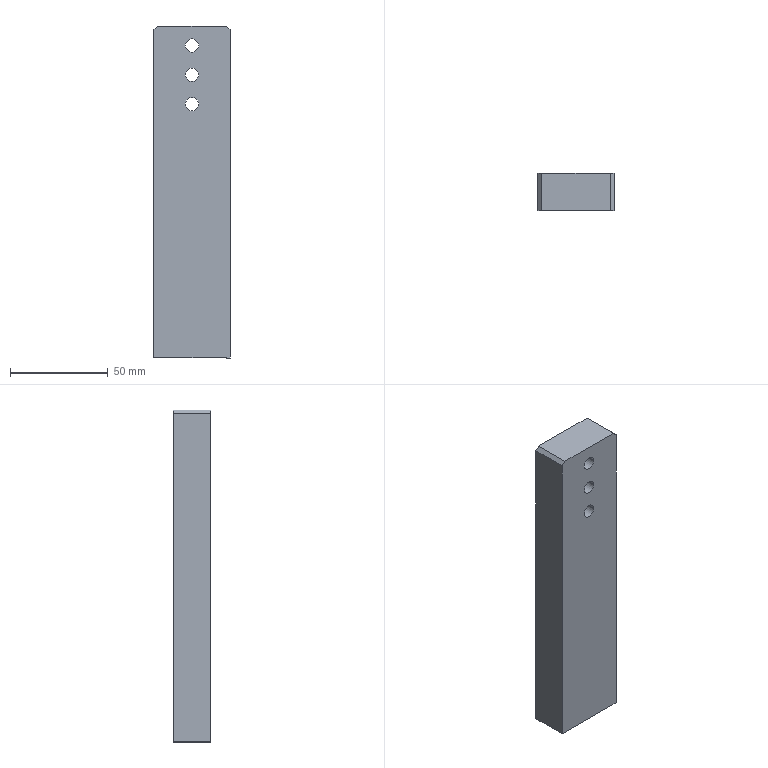Component | SolidWorks | FixedBlock-1 | 1 solid | 22 faces | box 39 x 19 x 170 mm | volume 123215 mm3 | cylinder 10 | plane 8 | cone 4 | commonest cylinder face diameters 6.8 x6 5 x4
build123d program:
from build123d import *

# Parameters (mm, degrees)
SKETCH2_W             = 39
SKETCH2_H             = 170
BOSS_EXTRUDE1_DEPTH   = 19
M6_TAPPED_HOLE1_D     = 5
M6_TAPPED_HOLE1_DEPTH = 15
M6_TAPPED_HOLE1_TIP   = 1.502
M8_TAPPED_HOLE1_D     = 6.8
M8_TAPPED_HOLE1_DEPTH = 19.75
M8_TAPPED_HOLE1_TIP   = 2.043
CHAMFER1_SIZE         = 2


with BuildPart() as part:
    # Sketch2 → Boss-Extrude1 (new body)
    with BuildSketch(Plane.XY):
        Rectangle(SKETCH2_W, SKETCH2_H)
    extrude(amount=BOSS_EXTRUDE1_DEPTH)

    # M6 Tapped Hole1
    with Locations(Plane(origin=(10, -85, 9.5), x_dir=(0, 0, -1), z_dir=(0, -1, 0))):
        with Locations((0, 0), (0, -20)):
            Hole(M6_TAPPED_HOLE1_D / 2, depth=M6_TAPPED_HOLE1_DEPTH)
            with Locations((0, 0, -(M6_TAPPED_HOLE1_DEPTH + M6_TAPPED_HOLE1_TIP / 2))):  # 118° drill point
                Cone(0, M6_TAPPED_HOLE1_D / 2, M6_TAPPED_HOLE1_TIP, mode=Mode.SUBTRACT)

    # M8 Tapped Hole1
    with Locations(Plane(origin=(0, 45, 19), x_dir=(1, 0, 0), z_dir=(0, 0, 1))):
        with Locations((0, 0), (0, 15), (0, 30)):
            Hole(M8_TAPPED_HOLE1_D / 2, depth=M8_TAPPED_HOLE1_DEPTH)
            with Locations((0, 0, -(M8_TAPPED_HOLE1_DEPTH + M8_TAPPED_HOLE1_TIP / 2))):  # 118° drill point
                Cone(0, M8_TAPPED_HOLE1_D / 2, M8_TAPPED_HOLE1_TIP, mode=Mode.SUBTRACT)

    # Chamfer1
    chamfer1_edges = [part.edges().sort_by_distance(p)[0] for p in [
        (-19.5, 85, 9.5),
        (19.5, 85, 9.5),
    ]]
    chamfer(chamfer1_edges, length=CHAMFER1_SIZE)


solid = part.part

# Placed as in the assembly
solid = solid.moved(Location((-48.047, 15.46, 106), (90, 0, 0)))
STEP:
#1=COLOUR_RGB('',0.7922,0.8196,0.9333);
#2=FILL_AREA_STYLE_COLOUR('',#1);
#3=FILL_AREA_STYLE('',(#2));
#4=SURFACE_STYLE_FILL_AREA(#3);
#5=SURFACE_SIDE_STYLE('',(#4));
#6=SURFACE_STYLE_USAGE(.BOTH.,#5);
#7=PRESENTATION_STYLE_ASSIGNMENT((#6));
#8=CARTESIAN_POINT('',(-1.758,0.6087,5.945));
#9=VERTEX_POINT('',#8);
#10=CARTESIAN_POINT('',(-2.025,0.6087,5.945));
#11=VERTEX_POINT('',#10);
#12=CARTESIAN_POINT('',(-1.892,0.6087,5.945));
#13=DIRECTION('',(-0.,1.,0.));
#14=DIRECTION('',(-1.,-0.,0.));
#15=AXIS2_PLACEMENT_3D('',#12,#13,#14);
#16=CIRCLE('',#15,0.1339);
#17=EDGE_CURVE('',#9,#11,#16,.T.);
#18=ORIENTED_EDGE('',*,*,#17,.T.);
#19=CARTESIAN_POINT('',(-2.025,-0.1394,5.945));
#20=VERTEX_POINT('',#19);
#21=CARTESIAN_POINT('',(-2.025,-0.1394,5.945));
#22=DIRECTION('',(0.,-1.,-0.));
#23=VECTOR('',#22,39.37);
#24=LINE('',#21,#23);
#25=EDGE_CURVE('',#11,#20,#24,.T.);
#26=ORIENTED_EDGE('',*,*,#25,.T.);
#27=CARTESIAN_POINT('',(-1.758,-0.1394,5.945));
#28=VERTEX_POINT('',#27);
#29=CARTESIAN_POINT('',(-1.892,-0.1394,5.945));
#30=DIRECTION('',(0.,-1.,-0.));
#31=DIRECTION('',(1.,0.,-0.));
#32=AXIS2_PLACEMENT_3D('',#29,#30,#31);
#33=CIRCLE('',#32,0.1339);
#34=EDGE_CURVE('',#20,#28,#33,.T.);
#35=ORIENTED_EDGE('',*,*,#34,.T.);
#36=CARTESIAN_POINT('',(-1.758,-0.1394,5.945));
#37=DIRECTION('',(0.,-1.,-0.));
#38=VECTOR('',#37,39.37);
#39=LINE('',#36,#38);
#40=EDGE_CURVE('',#9,#28,#39,.T.);
#41=ORIENTED_EDGE('',*,*,#40,.F.);
#42=EDGE_LOOP('',(#18,#26,#35,#41));
#43=FACE_OUTER_BOUND('',#42,.T.);
#44=CARTESIAN_POINT('',(-1.892,-0.1394,5.945));
#45=DIRECTION('',(0.,-1.,-0.));
#46=DIRECTION('',(1.,0.,-0.));
#47=AXIS2_PLACEMENT_3D('',#44,#45,#46);
#48=CYLINDRICAL_SURFACE('',#47,0.1339);
#49=ADVANCED_FACE('',(#43),#48,.F.);
#50=CARTESIAN_POINT('',(-1.758,0.6087,6.535));
#51=VERTEX_POINT('',#50);
#52=CARTESIAN_POINT('',(-2.025,0.6087,6.535));
#53=VERTEX_POINT('',#52);
#54=CARTESIAN_POINT('',(-1.892,0.6087,6.535));
#55=DIRECTION('',(-0.,1.,0.));
#56=DIRECTION('',(-1.,-0.,0.));
#57=AXIS2_PLACEMENT_3D('',#54,#55,#56);
#58=CIRCLE('',#57,0.1339);
#59=EDGE_CURVE('',#51,#53,#58,.T.);
#60=ORIENTED_EDGE('',*,*,#59,.T.);
#61=CARTESIAN_POINT('',(-2.025,-0.1394,6.535));
#62=VERTEX_POINT('',#61);
#63=CARTESIAN_POINT('',(-2.025,-0.1394,6.535));
#64=DIRECTION('',(0.,-1.,-0.));
#65=VECTOR('',#64,39.37);
#66=LINE('',#63,#65);
#67=EDGE_CURVE('',#53,#62,#66,.T.);
#68=ORIENTED_EDGE('',*,*,#67,.T.);
#69=CARTESIAN_POINT('',(-1.758,-0.1394,6.535));
#70=VERTEX_POINT('',#69);
#71=CARTESIAN_POINT('',(-1.892,-0.1394,6.535));
#72=DIRECTION('',(0.,-1.,-0.));
#73=DIRECTION('',(1.,0.,-0.));
#74=AXIS2_PLACEMENT_3D('',#71,#72,#73);
#75=CIRCLE('',#74,0.1339);
#76=EDGE_CURVE('',#62,#70,#75,.T.);
#77=ORIENTED_EDGE('',*,*,#76,.T.);
#78=CARTESIAN_POINT('',(-1.758,-0.1394,6.535));
#79=DIRECTION('',(0.,-1.,-0.));
#80=VECTOR('',#79,39.37);
#81=LINE('',#78,#80);
#82=EDGE_CURVE('',#51,#70,#81,.T.);
#83=ORIENTED_EDGE('',*,*,#82,.F.);
#84=EDGE_LOOP('',(#60,#68,#77,#83));
#85=FACE_OUTER_BOUND('',#84,.T.);
#86=CARTESIAN_POINT('',(-1.892,-0.1394,6.535));
#87=DIRECTION('',(0.,-1.,-0.));
#88=DIRECTION('',(1.,0.,-0.));
#89=AXIS2_PLACEMENT_3D('',#86,#87,#88);
#90=CYLINDRICAL_SURFACE('',#89,0.1339);
#91=ADVANCED_FACE('',(#85),#90,.F.);
#92=CARTESIAN_POINT('',(-1.758,0.6087,7.126));
#93=VERTEX_POINT('',#92);
#94=CARTESIAN_POINT('',(-2.025,0.6087,7.126));
#95=VERTEX_POINT('',#94);
#96=CARTESIAN_POINT('',(-1.892,0.6087,7.126));
#97=DIRECTION('',(-0.,1.,0.));
#98=DIRECTION('',(-1.,-0.,0.));
#99=AXIS2_PLACEMENT_3D('',#96,#97,#98);
#100=CIRCLE('',#99,0.1339);
#101=EDGE_CURVE('',#93,#95,#100,.T.);
#102=ORIENTED_EDGE('',*,*,#101,.T.);
#103=CARTESIAN_POINT('',(-2.025,-0.1394,7.126));
#104=VERTEX_POINT('',#103);
#105=CARTESIAN_POINT('',(-2.025,-0.1394,7.126));
#106=DIRECTION('',(0.,-1.,-0.));
#107=VECTOR('',#106,39.37);
#108=LINE('',#105,#107);
#109=EDGE_CURVE('',#95,#104,#108,.T.);
#110=ORIENTED_EDGE('',*,*,#109,.T.);
#111=CARTESIAN_POINT('',(-1.758,-0.1394,7.126));
#112=VERTEX_POINT('',#111);
#113=CARTESIAN_POINT('',(-1.892,-0.1394,7.126));
#114=DIRECTION('',(0.,-1.,-0.));
#115=DIRECTION('',(1.,0.,-0.));
#116=AXIS2_PLACEMENT_3D('',#113,#114,#115);
#117=CIRCLE('',#116,0.1339);
#118=EDGE_CURVE('',#104,#112,#117,.T.);
#119=ORIENTED_EDGE('',*,*,#118,.T.);
#120=CARTESIAN_POINT('',(-1.758,-0.1394,7.126));
#121=DIRECTION('',(0.,-1.,-0.));
#122=VECTOR('',#121,39.37);
#123=LINE('',#120,#122);
#124=EDGE_CURVE('',#93,#112,#123,.T.);
#125=ORIENTED_EDGE('',*,*,#124,.F.);
#126=EDGE_LOOP('',(#102,#110,#119,#125));
#127=FACE_OUTER_BOUND('',#126,.T.);
#128=CARTESIAN_POINT('',(-1.892,-0.1394,7.126));
#129=DIRECTION('',(0.,-1.,-0.));
#130=DIRECTION('',(1.,0.,-0.));
#131=AXIS2_PLACEMENT_3D('',#128,#129,#130);
#132=CYLINDRICAL_SURFACE('',#131,0.1339);
#133=ADVANCED_FACE('',(#127),#132,.F.);
#134=CARTESIAN_POINT('',(-1.498,0.1362,1.417));
#135=VERTEX_POINT('',#134);
#136=CARTESIAN_POINT('',(-1.498,0.3331,1.417));
#137=VERTEX_POINT('',#136);
#138=CARTESIAN_POINT('',(-1.498,0.2347,1.417));
#139=DIRECTION('',(-0.,0.,-1.));
#140=DIRECTION('',(0.,1.,0.));
#141=AXIS2_PLACEMENT_3D('',#138,#139,#140);
#142=CIRCLE('',#141,0.09843);
#143=EDGE_CURVE('',#135,#137,#142,.T.);
#144=ORIENTED_EDGE('',*,*,#143,.F.);
#145=CARTESIAN_POINT('',(-1.498,0.1362,0.8268));
#146=VERTEX_POINT('',#145);
#147=CARTESIAN_POINT('',(-1.498,0.1362,0.8268));
#148=DIRECTION('',(-0.,0.,-1.));
#149=VECTOR('',#148,39.37);
#150=LINE('',#147,#149);
#151=EDGE_CURVE('',#135,#146,#150,.T.);
#152=ORIENTED_EDGE('',*,*,#151,.T.);
#153=CARTESIAN_POINT('',(-1.498,0.3331,0.8268));
#154=VERTEX_POINT('',#153);
#155=CARTESIAN_POINT('',(-1.498,0.2347,0.8268));
#156=DIRECTION('',(-0.,0.,-1.));
#157=DIRECTION('',(0.,1.,0.));
#158=AXIS2_PLACEMENT_3D('',#155,#156,#157);
#159=CIRCLE('',#158,0.09843);
#160=EDGE_CURVE('',#146,#154,#159,.T.);
#161=ORIENTED_EDGE('',*,*,#160,.T.);
#162=CARTESIAN_POINT('',(-1.498,0.3331,0.8268));
#163=DIRECTION('',(-0.,0.,-1.));
#164=VECTOR('',#163,39.37);
#165=LINE('',#162,#164);
#166=EDGE_CURVE('',#137,#154,#165,.T.);
#167=ORIENTED_EDGE('',*,*,#166,.F.);
#168=EDGE_LOOP('',(#144,#152,#161,#167));
#169=FACE_OUTER_BOUND('',#168,.T.);
#170=CARTESIAN_POINT('',(-1.498,0.2347,0.8268));
#171=DIRECTION('',(-0.,0.,-1.));
#172=DIRECTION('',(0.,1.,0.));
#173=AXIS2_PLACEMENT_3D('',#170,#171,#172);
#174=CYLINDRICAL_SURFACE('',#173,0.09843);
#175=ADVANCED_FACE('',(#169),#174,.F.);
#176=CARTESIAN_POINT('',(-1.498,0.2347,1.476));
#177=VERTEX_POINT('',#176);
#178=CARTESIAN_POINT('',(-1.498,0.3331,1.417));
#179=DIRECTION('',(-0.,0.8572,-0.515));
#180=VECTOR('',#179,39.37);
#181=LINE('',#178,#180);
#182=EDGE_CURVE('',#177,#137,#181,.T.);
#183=ORIENTED_EDGE('',*,*,#182,.F.);
#184=CARTESIAN_POINT('',(-1.498,0.1362,1.417));
#185=DIRECTION('',(-0.,-0.8572,-0.515));
#186=VECTOR('',#185,39.37);
#187=LINE('',#184,#186);
#188=EDGE_CURVE('',#177,#135,#187,.T.);
#189=ORIENTED_EDGE('',*,*,#188,.T.);
#190=ORIENTED_EDGE('',*,*,#143,.T.);
#191=EDGE_LOOP('',(#183,#189,#190));
#192=FACE_OUTER_BOUND('',#191,.T.);
#193=CARTESIAN_POINT('',(-1.498,0.2347,1.417));
#194=DIRECTION('',(-0.,0.,-1.));
#195=DIRECTION('',(0.,1.,0.));
#196=AXIS2_PLACEMENT_3D('',#193,#194,#195);
#197=CONICAL_SURFACE('',#196,0.09843,1.03);
#198=ADVANCED_FACE('',(#192),#197,.F.);
#199=CARTESIAN_POINT('',(-2.285,0.1362,1.417));
#200=VERTEX_POINT('',#199);
#201=CARTESIAN_POINT('',(-2.285,0.3331,1.417));
#202=VERTEX_POINT('',#201);
#203=CARTESIAN_POINT('',(-2.285,0.2347,1.417));
#204=DIRECTION('',(-0.,0.,-1.));
#205=DIRECTION('',(0.,1.,0.));
#206=AXIS2_PLACEMENT_3D('',#203,#204,#205);
#207=CIRCLE('',#206,0.09843);
#208=EDGE_CURVE('',#200,#202,#207,.T.);
#209=ORIENTED_EDGE('',*,*,#208,.F.);
#210=CARTESIAN_POINT('',(-2.285,0.1362,0.8268));
#211=VERTEX_POINT('',#210);
#212=CARTESIAN_POINT('',(-2.285,0.1362,0.8268));
#213=DIRECTION('',(-0.,0.,-1.));
#214=VECTOR('',#213,39.37);
#215=LINE('',#212,#214);
#216=EDGE_CURVE('',#200,#211,#215,.T.);
#217=ORIENTED_EDGE('',*,*,#216,.T.);
#218=CARTESIAN_POINT('',(-2.285,0.3331,0.8268));
#219=VERTEX_POINT('',#218);
#220=CARTESIAN_POINT('',(-2.285,0.2347,0.8268));
#221=DIRECTION('',(-0.,0.,-1.));
#222=DIRECTION('',(0.,1.,0.));
#223=AXIS2_PLACEMENT_3D('',#220,#221,#222);
#224=CIRCLE('',#223,0.09843);
#225=EDGE_CURVE('',#211,#219,#224,.T.);
#226=ORIENTED_EDGE('',*,*,#225,.T.);
#227=CARTESIAN_POINT('',(-2.285,0.3331,0.8268));
#228=DIRECTION('',(-0.,0.,-1.));
#229=VECTOR('',#228,39.37);
#230=LINE('',#227,#229);
#231=EDGE_CURVE('',#202,#219,#230,.T.);
#232=ORIENTED_EDGE('',*,*,#231,.F.);
#233=EDGE_LOOP('',(#209,#217,#226,#232));
#234=FACE_OUTER_BOUND('',#233,.T.);
#235=CARTESIAN_POINT('',(-2.285,0.2347,0.8268));
#236=DIRECTION('',(-0.,0.,-1.));
#237=DIRECTION('',(0.,1.,0.));
#238=AXIS2_PLACEMENT_3D('',#235,#236,#237);
#239=CYLINDRICAL_SURFACE('',#238,0.09843);
#240=ADVANCED_FACE('',(#234),#239,.F.);
#241=CARTESIAN_POINT('',(-2.285,0.2347,1.476));
#242=VERTEX_POINT('',#241);
#243=CARTESIAN_POINT('',(-2.285,0.3331,1.417));
#244=DIRECTION('',(-0.,0.8572,-0.515));
#245=VECTOR('',#244,39.37);
#246=LINE('',#243,#245);
#247=EDGE_CURVE('',#242,#202,#246,.T.);
#248=ORIENTED_EDGE('',*,*,#247,.F.);
#249=CARTESIAN_POINT('',(-2.285,0.1362,1.417));
#250=DIRECTION('',(-0.,-0.8572,-0.515));
#251=VECTOR('',#250,39.37);
#252=LINE('',#249,#251);
#253=EDGE_CURVE('',#242,#200,#252,.T.);
#254=ORIENTED_EDGE('',*,*,#253,.T.);
#255=ORIENTED_EDGE('',*,*,#208,.T.);
#256=EDGE_LOOP('',(#248,#254,#255));
#257=FACE_OUTER_BOUND('',#256,.T.);
#258=CARTESIAN_POINT('',(-2.285,0.2347,1.417));
#259=DIRECTION('',(-0.,0.,-1.));
#260=DIRECTION('',(0.,1.,0.));
#261=AXIS2_PLACEMENT_3D('',#258,#259,#260);
#262=CONICAL_SURFACE('',#261,0.09843,1.03);
#263=ADVANCED_FACE('',(#257),#262,.F.);
#264=CARTESIAN_POINT('',(-1.124,0.6087,0.8268));
#265=VERTEX_POINT('',#264);
#266=CARTESIAN_POINT('',(-1.124,0.6087,7.441));
#267=VERTEX_POINT('',#266);
#268=CARTESIAN_POINT('',(-1.124,0.6087,0.8268));
#269=DIRECTION('',(0.,-0.,1.));
#270=VECTOR('',#269,39.37);
#271=LINE('',#268,#270);
#272=EDGE_CURVE('',#265,#267,#271,.T.);
#273=ORIENTED_EDGE('',*,*,#272,.T.);
#274=CARTESIAN_POINT('',(-1.124,-0.1394,7.441));
#275=VERTEX_POINT('',#274);
#276=CARTESIAN_POINT('',(-1.124,-0.1394,7.441));
#277=DIRECTION('',(0.,-1.,-0.));
#278=VECTOR('',#277,39.37);
#279=LINE('',#276,#278);
#280=EDGE_CURVE('',#267,#275,#279,.T.);
#281=ORIENTED_EDGE('',*,*,#280,.T.);
#282=CARTESIAN_POINT('',(-1.124,-0.1394,0.8268));
#283=VERTEX_POINT('',#282);
#284=CARTESIAN_POINT('',(-1.124,-0.1394,0.8268));
#285=DIRECTION('',(0.,-0.,1.));
#286=VECTOR('',#285,39.37);
#287=LINE('',#284,#286);
#288=EDGE_CURVE('',#283,#275,#287,.T.);
#289=ORIENTED_EDGE('',*,*,#288,.F.);
#290=CARTESIAN_POINT('',(-1.124,-0.1394,0.8268));
#291=DIRECTION('',(-0.,1.,0.));
#292=VECTOR('',#291,39.37);
#293=LINE('',#290,#292);
#294=EDGE_CURVE('',#283,#265,#293,.T.);
#295=ORIENTED_EDGE('',*,*,#294,.T.);
#296=EDGE_LOOP('',(#273,#281,#289,#295));
#297=FACE_OUTER_BOUND('',#296,.T.);
#298=CARTESIAN_POINT('',(-1.124,-0.1394,0.8268));
#299=DIRECTION('',(-1.,-0.,0.));
#300=DIRECTION('',(0.,-1.,-0.));
#301=AXIS2_PLACEMENT_3D('',#298,#299,#300);
#302=PLANE('',#301);
#303=ADVANCED_FACE('',(#297),#302,.F.);
#304=CARTESIAN_POINT('',(-1.203,-0.1394,7.52));
#305=VERTEX_POINT('',#304);
#306=CARTESIAN_POINT('',(-2.581,-0.1394,7.52));
#307=VERTEX_POINT('',#306);
#308=CARTESIAN_POINT('',(-2.659,-0.1394,7.52));
#309=DIRECTION('',(-1.,-0.,0.));
#310=VECTOR('',#309,39.37);
#311=LINE('',#308,#310);
#312=EDGE_CURVE('',#305,#307,#311,.T.);
#313=ORIENTED_EDGE('',*,*,#312,.F.);
#314=CARTESIAN_POINT('',(-1.203,0.6087,7.52));
#315=VERTEX_POINT('',#314);
#316=CARTESIAN_POINT('',(-1.203,-0.1394,7.52));
#317=DIRECTION('',(-0.,1.,0.));
#318=VECTOR('',#317,39.37);
#319=LINE('',#316,#318);
#320=EDGE_CURVE('',#305,#315,#319,.T.);
#321=ORIENTED_EDGE('',*,*,#320,.T.);
#322=CARTESIAN_POINT('',(-2.581,0.6087,7.52));
#323=VERTEX_POINT('',#322);
#324=CARTESIAN_POINT('',(-2.659,0.6087,7.52));
#325=DIRECTION('',(-1.,-0.,0.));
#326=VECTOR('',#325,39.37);
#327=LINE('',#324,#326);
#328=EDGE_CURVE('',#315,#323,#327,.T.);
#329=ORIENTED_EDGE('',*,*,#328,.T.);
#330=CARTESIAN_POINT('',(-2.581,-0.1394,7.52));
#331=DIRECTION('',(0.,-1.,-0.));
#332=VECTOR('',#331,39.37);
#333=LINE('',#330,#332);
#334=EDGE_CURVE('',#323,#307,#333,.T.);
#335=ORIENTED_EDGE('',*,*,#334,.T.);
#336=EDGE_LOOP('',(#313,#321,#329,#335));
#337=FACE_OUTER_BOUND('',#336,.T.);
#338=CARTESIAN_POINT('',(-2.659,-0.1394,7.52));
#339=DIRECTION('',(-0.,0.,-1.));
#340=DIRECTION('',(-0.,1.,0.));
#341=AXIS2_PLACEMENT_3D('',#338,#339,#340);
#342=PLANE('',#341);
#343=ADVANCED_FACE('',(#337),#342,.F.);
#344=CARTESIAN_POINT('',(-2.659,-0.1394,7.441));
#345=VERTEX_POINT('',#344);
#346=CARTESIAN_POINT('',(-2.659,-0.1394,0.8268));
#347=VERTEX_POINT('',#346);
#348=CARTESIAN_POINT('',(-2.659,-0.1394,0.8268));
#349=DIRECTION('',(-0.,0.,-1.));
#350=VECTOR('',#349,39.37);
#351=LINE('',#348,#350);
#352=EDGE_CURVE('',#345,#347,#351,.T.);
#353=ORIENTED_EDGE('',*,*,#352,.F.);
#354=CARTESIAN_POINT('',(-2.659,0.6087,7.441));
#355=VERTEX_POINT('',#354);
#356=CARTESIAN_POINT('',(-2.659,-0.1394,7.441));
#357=DIRECTION('',(-0.,1.,0.));
#358=VECTOR('',#357,39.37);
#359=LINE('',#356,#358);
#360=EDGE_CURVE('',#345,#355,#359,.T.);
#361=ORIENTED_EDGE('',*,*,#360,.T.);
#362=CARTESIAN_POINT('',(-2.659,0.6087,0.8268));
#363=VERTEX_POINT('',#362);
#364=CARTESIAN_POINT('',(-2.659,0.6087,0.8268));
#365=DIRECTION('',(-0.,0.,-1.));
#366=VECTOR('',#365,39.37);
#367=LINE('',#364,#366);
#368=EDGE_CURVE('',#355,#363,#367,.T.);
#369=ORIENTED_EDGE('',*,*,#368,.T.);
#370=CARTESIAN_POINT('',(-2.659,-0.1394,0.8268));
#371=DIRECTION('',(-0.,1.,0.));
#372=VECTOR('',#371,39.37);
#373=LINE('',#370,#372);
#374=EDGE_CURVE('',#347,#363,#373,.T.);
#375=ORIENTED_EDGE('',*,*,#374,.F.);
#376=EDGE_LOOP('',(#353,#361,#369,#375));
#377=FACE_OUTER_BOUND('',#376,.T.);
#378=CARTESIAN_POINT('',(-2.659,-0.1394,0.8268));
#379=DIRECTION('',(1.,0.,-0.));
#380=DIRECTION('',(-0.,1.,0.));
#381=AXIS2_PLACEMENT_3D('',#378,#379,#380);
#382=PLANE('',#381);
#383=ADVANCED_FACE('',(#377),#382,.F.);
#384=CARTESIAN_POINT('',(-1.498,0.2347,0.8268));
#385=DIRECTION('',(-0.,0.,-1.));
#386=DIRECTION('',(0.,1.,0.));
#387=AXIS2_PLACEMENT_3D('',#384,#385,#386);
#388=CIRCLE('',#387,0.09843);
#389=EDGE_CURVE('',#154,#146,#388,.T.);
#390=ORIENTED_EDGE('',*,*,#389,.F.);
#391=ORIENTED_EDGE('',*,*,#160,.F.);
#392=EDGE_LOOP('',(#390,#391));
#393=FACE_BOUND('',#392,.T.);
#394=CARTESIAN_POINT('',(-2.285,0.2347,0.8268));
#395=DIRECTION('',(-0.,0.,-1.));
#396=DIRECTION('',(0.,1.,0.));
#397=AXIS2_PLACEMENT_3D('',#394,#395,#396);
#398=CIRCLE('',#397,0.09843);
#399=EDGE_CURVE('',#219,#211,#398,.T.);
#400=ORIENTED_EDGE('',*,*,#399,.F.);
#401=ORIENTED_EDGE('',*,*,#225,.F.);
#402=EDGE_LOOP('',(#400,#401));
#403=FACE_BOUND('',#402,.T.);
#404=CARTESIAN_POINT('',(-2.659,0.6087,0.8268));
#405=DIRECTION('',(1.,0.,-0.));
#406=VECTOR('',#405,39.37);
#407=LINE('',#404,#406);
#408=EDGE_CURVE('',#363,#265,#407,.T.);
#409=ORIENTED_EDGE('',*,*,#408,.T.);
#410=ORIENTED_EDGE('',*,*,#294,.F.);
#411=CARTESIAN_POINT('',(-2.659,-0.1394,0.8268));
#412=DIRECTION('',(1.,0.,-0.));
#413=VECTOR('',#412,39.37);
#414=LINE('',#411,#413);
#415=EDGE_CURVE('',#347,#283,#414,.T.);
#416=ORIENTED_EDGE('',*,*,#415,.F.);
#417=ORIENTED_EDGE('',*,*,#374,.T.);
#418=EDGE_LOOP('',(#409,#410,#416,#417));
#419=FACE_OUTER_BOUND('',#418,.T.);
#420=CARTESIAN_POINT('',(-2.659,-0.1394,0.8268));
#421=DIRECTION('',(0.,-0.,1.));
#422=DIRECTION('',(0.,-1.,-0.));
#423=AXIS2_PLACEMENT_3D('',#420,#421,#422);
#424=PLANE('',#423);
#425=ADVANCED_FACE('',(#393,#403,#419),#424,.F.);
#426=CARTESIAN_POINT('',(-1.892,-0.1394,5.945));
#427=DIRECTION('',(0.,-1.,-0.));
#428=DIRECTION('',(1.,0.,-0.));
#429=AXIS2_PLACEMENT_3D('',#426,#427,#428);
#430=CIRCLE('',#429,0.1339);
#431=EDGE_CURVE('',#28,#20,#430,.T.);
#432=ORIENTED_EDGE('',*,*,#431,.F.);
#433=ORIENTED_EDGE('',*,*,#34,.F.);
#434=EDGE_LOOP('',(#432,#433));
#435=FACE_BOUND('',#434,.T.);
#436=CARTESIAN_POINT('',(-1.892,-0.1394,6.535));
#437=DIRECTION('',(0.,-1.,-0.));
#438=DIRECTION('',(1.,0.,-0.));
#439=AXIS2_PLACEMENT_3D('',#436,#437,#438);
#440=CIRCLE('',#439,0.1339);
#441=EDGE_CURVE('',#70,#62,#440,.T.);
#442=ORIENTED_EDGE('',*,*,#441,.F.);
#443=ORIENTED_EDGE('',*,*,#76,.F.);
#444=EDGE_LOOP('',(#442,#443));
#445=FACE_BOUND('',#444,.T.);
#446=CARTESIAN_POINT('',(-1.892,-0.1394,7.126));
#447=DIRECTION('',(0.,-1.,-0.));
#448=DIRECTION('',(1.,0.,-0.));
#449=AXIS2_PLACEMENT_3D('',#446,#447,#448);
#450=CIRCLE('',#449,0.1339);
#451=EDGE_CURVE('',#112,#104,#450,.T.);
#452=ORIENTED_EDGE('',*,*,#451,.F.);
#453=ORIENTED_EDGE('',*,*,#118,.F.);
#454=EDGE_LOOP('',(#452,#453));
#455=FACE_BOUND('',#454,.T.);
#456=ORIENTED_EDGE('',*,*,#288,.T.);
#457=CARTESIAN_POINT('',(-1.203,-0.1394,7.52));
#458=DIRECTION('',(-0.7071,-0.,0.7071));
#459=VECTOR('',#458,39.37);
#460=LINE('',#457,#459);
#461=EDGE_CURVE('',#275,#305,#460,.T.);
#462=ORIENTED_EDGE('',*,*,#461,.T.);
#463=ORIENTED_EDGE('',*,*,#312,.T.);
#464=CARTESIAN_POINT('',(-2.659,-0.1394,7.441));
#465=DIRECTION('',(-0.7071,-0.,-0.7071));
#466=VECTOR('',#465,39.37);
#467=LINE('',#464,#466);
#468=EDGE_CURVE('',#307,#345,#467,.T.);
#469=ORIENTED_EDGE('',*,*,#468,.T.);
#470=ORIENTED_EDGE('',*,*,#352,.T.);
#471=ORIENTED_EDGE('',*,*,#415,.T.);
#472=EDGE_LOOP('',(#456,#462,#463,#469,#470,#471));
#473=FACE_OUTER_BOUND('',#472,.T.);
#474=CARTESIAN_POINT('',(-1.892,-0.1394,4.173));
#475=DIRECTION('',(-0.,1.,0.));
#476=DIRECTION('',(-1.,-0.,0.));
#477=AXIS2_PLACEMENT_3D('',#474,#475,#476);
#478=PLANE('',#477);
#479=ADVANCED_FACE('',(#435,#445,#455,#473),#478,.F.);
#480=ORIENTED_EDGE('',*,*,#17,.F.);
#481=CARTESIAN_POINT('',(-1.892,0.6087,5.945));
#482=DIRECTION('',(-0.,1.,0.));
#483=DIRECTION('',(-1.,-0.,0.));
#484=AXIS2_PLACEMENT_3D('',#481,#482,#483);
#485=CIRCLE('',#484,0.1339);
#486=EDGE_CURVE('',#11,#9,#485,.T.);
#487=ORIENTED_EDGE('',*,*,#486,.F.);
#488=EDGE_LOOP('',(#480,#487));
#489=FACE_BOUND('',#488,.T.);
#490=ORIENTED_EDGE('',*,*,#59,.F.);
#491=CARTESIAN_POINT('',(-1.892,0.6087,6.535));
#492=DIRECTION('',(-0.,1.,0.));
#493=DIRECTION('',(-1.,-0.,0.));
#494=AXIS2_PLACEMENT_3D('',#491,#492,#493);
#495=CIRCLE('',#494,0.1339);
#496=EDGE_CURVE('',#53,#51,#495,.T.);
#497=ORIENTED_EDGE('',*,*,#496,.F.);
#498=EDGE_LOOP('',(#490,#497));
#499=FACE_BOUND('',#498,.T.);
#500=ORIENTED_EDGE('',*,*,#101,.F.);
#501=CARTESIAN_POINT('',(-1.892,0.6087,7.126));
#502=DIRECTION('',(-0.,1.,0.));
#503=DIRECTION('',(-1.,-0.,0.));
#504=AXIS2_PLACEMENT_3D('',#501,#502,#503);
#505=CIRCLE('',#504,0.1339);
#506=EDGE_CURVE('',#95,#93,#505,.T.);
#507=ORIENTED_EDGE('',*,*,#506,.F.);
#508=EDGE_LOOP('',(#500,#507));
#509=FACE_BOUND('',#508,.T.);
#510=ORIENTED_EDGE('',*,*,#328,.F.);
#511=CARTESIAN_POINT('',(0.1261,0.6087,6.191));
#512=DIRECTION('',(0.7071,0.,-0.7071));
#513=VECTOR('',#512,39.37);
#514=LINE('',#511,#513);
#515=EDGE_CURVE('',#315,#267,#514,.T.);
#516=ORIENTED_EDGE('',*,*,#515,.T.);
#517=ORIENTED_EDGE('',*,*,#272,.F.);
#518=ORIENTED_EDGE('',*,*,#408,.F.);
#519=ORIENTED_EDGE('',*,*,#368,.F.);
#520=CARTESIAN_POINT('',(-3.909,0.6087,6.191));
#521=DIRECTION('',(0.7071,0.,0.7071));
#522=VECTOR('',#521,39.37);
#523=LINE('',#520,#522);
#524=EDGE_CURVE('',#355,#323,#523,.T.);
#525=ORIENTED_EDGE('',*,*,#524,.T.);
#526=EDGE_LOOP('',(#510,#516,#517,#518,#519,#525));
#527=FACE_OUTER_BOUND('',#526,.T.);
#528=CARTESIAN_POINT('',(-1.892,0.6087,4.173));
#529=DIRECTION('',(-0.,1.,0.));
#530=DIRECTION('',(-1.,-0.,0.));
#531=AXIS2_PLACEMENT_3D('',#528,#529,#530);
#532=PLANE('',#531);
#533=ADVANCED_FACE('',(#489,#499,#509,#527),#532,.T.);
#534=ORIENTED_EDGE('',*,*,#253,.F.);
#535=ORIENTED_EDGE('',*,*,#247,.T.);
#536=CARTESIAN_POINT('',(-2.285,0.2347,1.417));
#537=DIRECTION('',(-0.,0.,-1.));
#538=DIRECTION('',(0.,1.,0.));
#539=AXIS2_PLACEMENT_3D('',#536,#537,#538);
#540=CIRCLE('',#539,0.09843);
#541=EDGE_CURVE('',#202,#200,#540,.T.);
#542=ORIENTED_EDGE('',*,*,#541,.T.);
#543=EDGE_LOOP('',(#534,#535,#542));
#544=FACE_OUTER_BOUND('',#543,.T.);
#545=CARTESIAN_POINT('',(-2.285,0.2347,1.417));
#546=DIRECTION('',(-0.,0.,-1.));
#547=DIRECTION('',(0.,1.,0.));
#548=AXIS2_PLACEMENT_3D('',#545,#546,#547);
#549=CONICAL_SURFACE('',#548,0.09843,1.03);
#550=ADVANCED_FACE('',(#544),#549,.F.);
#551=ORIENTED_EDGE('',*,*,#216,.F.);
#552=ORIENTED_EDGE('',*,*,#541,.F.);
#553=ORIENTED_EDGE('',*,*,#231,.T.);
#554=ORIENTED_EDGE('',*,*,#399,.T.);
#555=EDGE_LOOP('',(#551,#552,#553,#554));
#556=FACE_OUTER_BOUND('',#555,.T.);
#557=CARTESIAN_POINT('',(-2.285,0.2347,0.8268));
#558=DIRECTION('',(-0.,0.,-1.));
#559=DIRECTION('',(0.,1.,0.));
#560=AXIS2_PLACEMENT_3D('',#557,#558,#559);
#561=CYLINDRICAL_SURFACE('',#560,0.09843);
#562=ADVANCED_FACE('',(#556),#561,.F.);
#563=ORIENTED_EDGE('',*,*,#188,.F.);
#564=ORIENTED_EDGE('',*,*,#182,.T.);
#565=CARTESIAN_POINT('',(-1.498,0.2347,1.417));
#566=DIRECTION('',(-0.,0.,-1.));
#567=DIRECTION('',(0.,1.,0.));
#568=AXIS2_PLACEMENT_3D('',#565,#566,#567);
#569=CIRCLE('',#568,0.09843);
#570=EDGE_CURVE('',#137,#135,#569,.T.);
#571=ORIENTED_EDGE('',*,*,#570,.T.);
#572=EDGE_LOOP('',(#563,#564,#571));
#573=FACE_OUTER_BOUND('',#572,.T.);
#574=CARTESIAN_POINT('',(-1.498,0.2347,1.417));
#575=DIRECTION('',(-0.,0.,-1.));
#576=DIRECTION('',(0.,1.,0.));
#577=AXIS2_PLACEMENT_3D('',#574,#575,#576);
#578=CONICAL_SURFACE('',#577,0.09843,1.03);
#579=ADVANCED_FACE('',(#573),#578,.F.);
#580=ORIENTED_EDGE('',*,*,#151,.F.);
#581=ORIENTED_EDGE('',*,*,#570,.F.);
#582=ORIENTED_EDGE('',*,*,#166,.T.);
#583=ORIENTED_EDGE('',*,*,#389,.T.);
#584=EDGE_LOOP('',(#580,#581,#582,#583));
#585=FACE_OUTER_BOUND('',#584,.T.);
#586=CARTESIAN_POINT('',(-1.498,0.2347,0.8268));
#587=DIRECTION('',(-0.,0.,-1.));
#588=DIRECTION('',(0.,1.,0.));
#589=AXIS2_PLACEMENT_3D('',#586,#587,#588);
#590=CYLINDRICAL_SURFACE('',#589,0.09843);
#591=ADVANCED_FACE('',(#585),#590,.F.);
#592=ORIENTED_EDGE('',*,*,#109,.F.);
#593=ORIENTED_EDGE('',*,*,#506,.T.);
#594=ORIENTED_EDGE('',*,*,#124,.T.);
#595=ORIENTED_EDGE('',*,*,#451,.T.);
#596=EDGE_LOOP('',(#592,#593,#594,#595));
#597=FACE_OUTER_BOUND('',#596,.T.);
#598=CARTESIAN_POINT('',(-1.892,-0.1394,7.126));
#599=DIRECTION('',(0.,-1.,-0.));
#600=DIRECTION('',(1.,0.,-0.));
#601=AXIS2_PLACEMENT_3D('',#598,#599,#600);
#602=CYLINDRICAL_SURFACE('',#601,0.1339);
#603=ADVANCED_FACE('',(#597),#602,.F.);
#604=ORIENTED_EDGE('',*,*,#67,.F.);
#605=ORIENTED_EDGE('',*,*,#496,.T.);
#606=ORIENTED_EDGE('',*,*,#82,.T.);
#607=ORIENTED_EDGE('',*,*,#441,.T.);
#608=EDGE_LOOP('',(#604,#605,#606,#607));
#609=FACE_OUTER_BOUND('',#608,.T.);
#610=CARTESIAN_POINT('',(-1.892,-0.1394,6.535));
#611=DIRECTION('',(0.,-1.,-0.));
#612=DIRECTION('',(1.,0.,-0.));
#613=AXIS2_PLACEMENT_3D('',#610,#611,#612);
#614=CYLINDRICAL_SURFACE('',#613,0.1339);
#615=ADVANCED_FACE('',(#609),#614,.F.);
#616=ORIENTED_EDGE('',*,*,#25,.F.);
#617=ORIENTED_EDGE('',*,*,#486,.T.);
#618=ORIENTED_EDGE('',*,*,#40,.T.);
#619=ORIENTED_EDGE('',*,*,#431,.T.);
#620=EDGE_LOOP('',(#616,#617,#618,#619));
#621=FACE_OUTER_BOUND('',#620,.T.);
#622=CARTESIAN_POINT('',(-1.892,-0.1394,5.945));
#623=DIRECTION('',(0.,-1.,-0.));
#624=DIRECTION('',(1.,0.,-0.));
#625=AXIS2_PLACEMENT_3D('',#622,#623,#624);
#626=CYLINDRICAL_SURFACE('',#625,0.1339);
#627=ADVANCED_FACE('',(#621),#626,.F.);
#628=ORIENTED_EDGE('',*,*,#461,.F.);
#629=ORIENTED_EDGE('',*,*,#280,.F.);
#630=ORIENTED_EDGE('',*,*,#515,.F.);
#631=ORIENTED_EDGE('',*,*,#320,.F.);
#632=EDGE_LOOP('',(#628,#629,#630,#631));
#633=FACE_OUTER_BOUND('',#632,.T.);
#634=CARTESIAN_POINT('',(-1.203,-0.1394,7.52));
#635=DIRECTION('',(-0.7071,-0.,-0.7071));
#636=DIRECTION('',(-0.,1.,0.));
#637=AXIS2_PLACEMENT_3D('',#634,#635,#636);
#638=PLANE('',#637);
#639=ADVANCED_FACE('',(#633),#638,.F.);
#640=ORIENTED_EDGE('',*,*,#468,.F.);
#641=ORIENTED_EDGE('',*,*,#334,.F.);
#642=ORIENTED_EDGE('',*,*,#524,.F.);
#643=ORIENTED_EDGE('',*,*,#360,.F.);
#644=EDGE_LOOP('',(#640,#641,#642,#643));
#645=FACE_OUTER_BOUND('',#644,.T.);
#646=CARTESIAN_POINT('',(-2.659,-0.1394,7.441));
#647=DIRECTION('',(0.7071,0.,-0.7071));
#648=DIRECTION('',(-0.,1.,0.));
#649=AXIS2_PLACEMENT_3D('',#646,#647,#648);
#650=PLANE('',#649);
#651=ADVANCED_FACE('',(#645),#650,.F.);
#652=CLOSED_SHELL('',(#49,#91,#133,#175,#198,#240,#263,#303,#343,#383,#425,#479,#533,#550,#562,#579,#591,#603,#615,#627,#639,#651));
#653=MANIFOLD_SOLID_BREP('',#652);
#654=STYLED_ITEM('',(#7),#653);
#655=(LENGTH_UNIT()NAMED_UNIT(*)SI_UNIT($,.METRE.));
#656=LENGTH_MEASURE_WITH_UNIT(LENGTH_MEASURE(0.0254),#655);
#657=DIMENSIONAL_EXPONENTS(1.,0.,0.,0.,0.,0.,0.);
#658=(CONVERSION_BASED_UNIT('',#656)LENGTH_UNIT()NAMED_UNIT(#657));
#659=UNCERTAINTY_MEASURE_WITH_UNIT(LENGTH_MEASURE(0.00001),#658,'','');
#660=(NAMED_UNIT(*)PLANE_ANGLE_UNIT()SI_UNIT($,.RADIAN.));
#661=(NAMED_UNIT(*)SI_UNIT($,.STERADIAN.)SOLID_ANGLE_UNIT());
#662=(GEOMETRIC_REPRESENTATION_CONTEXT(3)GLOBAL_UNCERTAINTY_ASSIGNED_CONTEXT((#659))GLOBAL_UNIT_ASSIGNED_CONTEXT((#658,#660,#661))REPRESENTATION_CONTEXT('',''));
#663=MECHANICAL_DESIGN_GEOMETRIC_PRESENTATION_REPRESENTATION('',(#654),#662);
#664=PRESENTATION_LAYER_ASSIGNMENT('','',(#654));
#665=CARTESIAN_POINT('',(0.,0.,0.));
#666=DIRECTION('',(0.,0.,1.));
#667=DIRECTION('',(1.,0.,0.));
#668=AXIS2_PLACEMENT_3D('',#665,#666,#667);
#669=(LENGTH_UNIT()NAMED_UNIT(*)SI_UNIT($,.METRE.));
#670=LENGTH_MEASURE_WITH_UNIT(LENGTH_MEASURE(0.0254),#669);
#671=DIMENSIONAL_EXPONENTS(1.,0.,0.,0.,0.,0.,0.);
#672=(CONVERSION_BASED_UNIT('',#670)LENGTH_UNIT()NAMED_UNIT(#671));
#673=UNCERTAINTY_MEASURE_WITH_UNIT(LENGTH_MEASURE(0.00001),#672,'','');
#674=(NAMED_UNIT(*)PLANE_ANGLE_UNIT()SI_UNIT($,.RADIAN.));
#675=(NAMED_UNIT(*)SI_UNIT($,.STERADIAN.)SOLID_ANGLE_UNIT());
#676=(GEOMETRIC_REPRESENTATION_CONTEXT(3)GLOBAL_UNCERTAINTY_ASSIGNED_CONTEXT((#673))GLOBAL_UNIT_ASSIGNED_CONTEXT((#672,#674,#675))REPRESENTATION_CONTEXT('',''));
#677=ADVANCED_BREP_SHAPE_REPRESENTATION('',(#653,#668),#676);